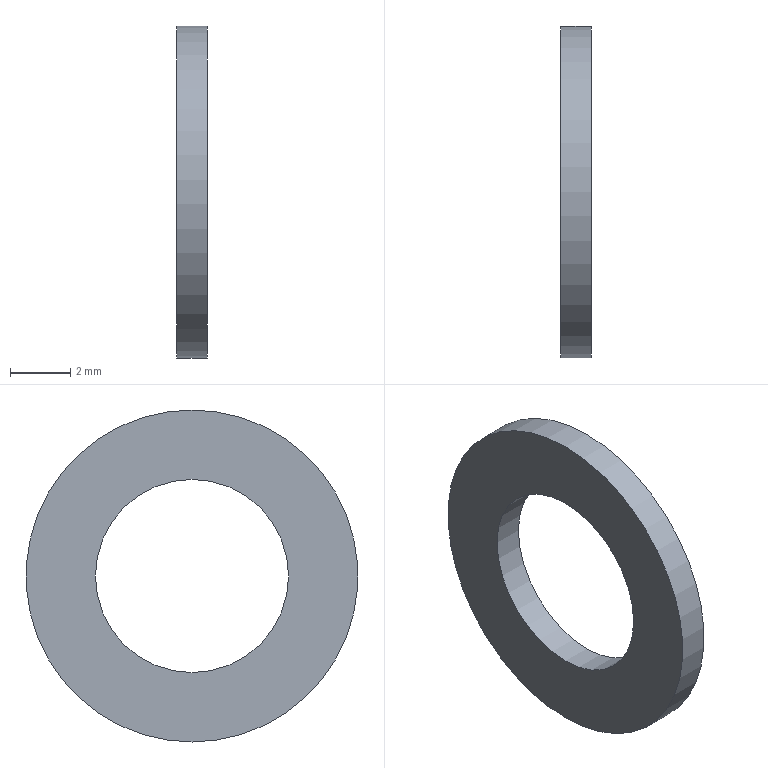Component | NX | ASSY_PRAC_PART_5 | 1 solid | 4 faces | box 1 x 11 x 11 mm | volume 63 mm3 | cylinder 2 | plane 2 | commonest cylinder face diameters 11 x1 6.4 x1
STEP:
#1=CARTESIAN_POINT('',(0.,0.,0.));
#2=DIRECTION('',(0.,0.,1.));
#3=DIRECTION('',(1.,0.,0.));
#4=AXIS2_PLACEMENT_3D('',#1,#2,#3);
#5=CARTESIAN_POINT('',(17.5,0.3851,26.061));
#6=VERTEX_POINT('',#5);
#7=CARTESIAN_POINT('',(17.5,0.3851,20.561));
#8=DIRECTION('',(-1.,0.,0.));
#9=DIRECTION('',(0.,0.,1.));
#10=AXIS2_PLACEMENT_3D('',#7,#8,#9);
#11=CIRCLE('',#10,5.5);
#12=CARTESIAN_POINT('',(17.5,0.3851,20.561));
#13=DIRECTION('',(1.,0.,0.));
#14=DIRECTION('',(0.,0.,-1.));
#15=AXIS2_PLACEMENT_3D('',#12,#13,#14);
#16=CYLINDRICAL_SURFACE('',#15,5.5);
#17=CARTESIAN_POINT('',(9.425,0.));
#18=DIRECTION('',(-1.,0.));
#19=VECTOR('',#18,1.);
#20=LINE('',#17,#19);
#21=(GEOMETRIC_REPRESENTATION_CONTEXT(2)PARAMETRIC_REPRESENTATION_CONTEXT()REPRESENTATION_CONTEXT('',''));
#22=DEFINITIONAL_REPRESENTATION('',(#20),#21);
#23=PCURVE('',#16,#22);
#24=CARTESIAN_POINT('',(17.5,0.3851,20.561));
#25=DIRECTION('',(-1.,0.,0.));
#26=DIRECTION('',(0.,0.,1.));
#27=AXIS2_PLACEMENT_3D('',#24,#25,#26);
#28=PLANE('',#27);
#29=CARTESIAN_POINT('',(0.,0.));
#30=DIRECTION('',(1.,0.));
#31=AXIS2_PLACEMENT_2D('',#29,#30);
#32=CIRCLE('',#31,5.5);
#33=(GEOMETRIC_REPRESENTATION_CONTEXT(2)PARAMETRIC_REPRESENTATION_CONTEXT()REPRESENTATION_CONTEXT('',''));
#34=DEFINITIONAL_REPRESENTATION('',(#32),#33);
#35=PCURVE('',#28,#34);
#36=SURFACE_CURVE('',#11,(#23,#35),.PCURVE_S1.);
#37=EDGE_CURVE('',#6,#6,#36,.T.);
#38=ORIENTED_EDGE('',*,*,#37,.F.);
#39=CARTESIAN_POINT('',(18.5,0.3851,26.061));
#40=VERTEX_POINT('',#39);
#41=CARTESIAN_POINT('',(17.5,0.3851,26.061));
#42=CARTESIAN_POINT('',(18.5,0.3851,26.061));
#43=B_SPLINE_CURVE_WITH_KNOTS('',1,(#41,#42),.UNSPECIFIED.,.F.,.F.,(2,2),(0.,1.),.PIECEWISE_BEZIER_KNOTS.);
#44=CARTESIAN_POINT('',(9.425,0.));
#45=DIRECTION('',(0.,1.));
#46=VECTOR('',#45,1.);
#47=LINE('',#44,#46);
#48=(GEOMETRIC_REPRESENTATION_CONTEXT(2)PARAMETRIC_REPRESENTATION_CONTEXT()REPRESENTATION_CONTEXT('',''));
#49=DEFINITIONAL_REPRESENTATION('',(#47),#48);
#50=PCURVE('',#16,#49);
#51=CARTESIAN_POINT('',(3.142,0.));
#52=DIRECTION('',(0.,1.));
#53=VECTOR('',#52,1.);
#54=LINE('',#51,#53);
#55=(GEOMETRIC_REPRESENTATION_CONTEXT(2)PARAMETRIC_REPRESENTATION_CONTEXT()REPRESENTATION_CONTEXT('',''));
#56=DEFINITIONAL_REPRESENTATION('',(#54),#55);
#57=PCURVE('',#16,#56);
#58=SEAM_CURVE('',#43,(#50,#57),.PCURVE_S1.);
#59=EDGE_CURVE('',#6,#40,#58,.T.);
#60=ORIENTED_EDGE('',*,*,#59,.T.);
#61=CARTESIAN_POINT('',(18.5,0.3851,20.561));
#62=DIRECTION('',(-1.,0.,0.));
#63=DIRECTION('',(0.,0.,1.));
#64=AXIS2_PLACEMENT_3D('',#61,#62,#63);
#65=CIRCLE('',#64,5.5);
#66=CARTESIAN_POINT('',(9.425,1.));
#67=DIRECTION('',(-1.,0.));
#68=VECTOR('',#67,1.);
#69=LINE('',#66,#68);
#70=(GEOMETRIC_REPRESENTATION_CONTEXT(2)PARAMETRIC_REPRESENTATION_CONTEXT()REPRESENTATION_CONTEXT('',''));
#71=DEFINITIONAL_REPRESENTATION('',(#69),#70);
#72=PCURVE('',#16,#71);
#73=CARTESIAN_POINT('',(18.5,0.3851,20.561));
#74=DIRECTION('',(-1.,0.,0.));
#75=DIRECTION('',(0.,0.,1.));
#76=AXIS2_PLACEMENT_3D('',#73,#74,#75);
#77=PLANE('',#76);
#78=CARTESIAN_POINT('',(0.,0.));
#79=DIRECTION('',(1.,0.));
#80=AXIS2_PLACEMENT_2D('',#78,#79);
#81=CIRCLE('',#80,5.5);
#82=(GEOMETRIC_REPRESENTATION_CONTEXT(2)PARAMETRIC_REPRESENTATION_CONTEXT()REPRESENTATION_CONTEXT('',''));
#83=DEFINITIONAL_REPRESENTATION('',(#81),#82);
#84=PCURVE('',#77,#83);
#85=SURFACE_CURVE('',#65,(#72,#84),.PCURVE_S1.);
#86=EDGE_CURVE('',#40,#40,#85,.T.);
#87=ORIENTED_EDGE('',*,*,#86,.T.);
#88=ORIENTED_EDGE('',*,*,#59,.F.);
#89=EDGE_LOOP('',(#38,#60,#87,#88));
#90=FACE_BOUND('',#89,.T.);
#91=ADVANCED_FACE('',(#90),#16,.T.);
#92=CARTESIAN_POINT('',(17.5,0.3851,23.761));
#93=VERTEX_POINT('',#92);
#94=CARTESIAN_POINT('',(17.5,0.3851,20.561));
#95=DIRECTION('',(-1.,0.,0.));
#96=DIRECTION('',(0.,0.,1.));
#97=AXIS2_PLACEMENT_3D('',#94,#95,#96);
#98=CIRCLE('',#97,3.2);
#99=CARTESIAN_POINT('',(17.5,0.3851,20.561));
#100=DIRECTION('',(1.,0.,0.));
#101=DIRECTION('',(0.,0.,-1.));
#102=AXIS2_PLACEMENT_3D('',#99,#100,#101);
#103=CYLINDRICAL_SURFACE('',#102,3.2);
#104=CARTESIAN_POINT('',(9.425,0.));
#105=DIRECTION('',(-1.,0.));
#106=VECTOR('',#105,1.);
#107=LINE('',#104,#106);
#108=(GEOMETRIC_REPRESENTATION_CONTEXT(2)PARAMETRIC_REPRESENTATION_CONTEXT()REPRESENTATION_CONTEXT('',''));
#109=DEFINITIONAL_REPRESENTATION('',(#107),#108);
#110=PCURVE('',#103,#109);
#111=CARTESIAN_POINT('',(0.,0.));
#112=DIRECTION('',(1.,0.));
#113=AXIS2_PLACEMENT_2D('',#111,#112);
#114=CIRCLE('',#113,3.2);
#115=(GEOMETRIC_REPRESENTATION_CONTEXT(2)PARAMETRIC_REPRESENTATION_CONTEXT()REPRESENTATION_CONTEXT('',''));
#116=DEFINITIONAL_REPRESENTATION('',(#114),#115);
#117=PCURVE('',#28,#116);
#118=SURFACE_CURVE('',#98,(#110,#117),.PCURVE_S1.);
#119=EDGE_CURVE('',#93,#93,#118,.T.);
#120=ORIENTED_EDGE('',*,*,#119,.F.);
#121=CARTESIAN_POINT('',(18.5,0.3851,23.761));
#122=VERTEX_POINT('',#121);
#123=CARTESIAN_POINT('',(17.5,0.3851,23.761));
#124=CARTESIAN_POINT('',(18.5,0.3851,23.761));
#125=B_SPLINE_CURVE_WITH_KNOTS('',1,(#123,#124),.UNSPECIFIED.,.F.,.F.,(2,2),(0.,1.),.PIECEWISE_BEZIER_KNOTS.);
#126=CARTESIAN_POINT('',(9.425,0.));
#127=DIRECTION('',(0.,1.));
#128=VECTOR('',#127,1.);
#129=LINE('',#126,#128);
#130=(GEOMETRIC_REPRESENTATION_CONTEXT(2)PARAMETRIC_REPRESENTATION_CONTEXT()REPRESENTATION_CONTEXT('',''));
#131=DEFINITIONAL_REPRESENTATION('',(#129),#130);
#132=PCURVE('',#103,#131);
#133=CARTESIAN_POINT('',(3.142,0.));
#134=DIRECTION('',(0.,1.));
#135=VECTOR('',#134,1.);
#136=LINE('',#133,#135);
#137=(GEOMETRIC_REPRESENTATION_CONTEXT(2)PARAMETRIC_REPRESENTATION_CONTEXT()REPRESENTATION_CONTEXT('',''));
#138=DEFINITIONAL_REPRESENTATION('',(#136),#137);
#139=PCURVE('',#103,#138);
#140=SEAM_CURVE('',#125,(#132,#139),.PCURVE_S1.);
#141=EDGE_CURVE('',#93,#122,#140,.T.);
#142=ORIENTED_EDGE('',*,*,#141,.T.);
#143=CARTESIAN_POINT('',(18.5,0.3851,20.561));
#144=DIRECTION('',(-1.,0.,0.));
#145=DIRECTION('',(0.,0.,1.));
#146=AXIS2_PLACEMENT_3D('',#143,#144,#145);
#147=CIRCLE('',#146,3.2);
#148=CARTESIAN_POINT('',(9.425,1.));
#149=DIRECTION('',(-1.,0.));
#150=VECTOR('',#149,1.);
#151=LINE('',#148,#150);
#152=(GEOMETRIC_REPRESENTATION_CONTEXT(2)PARAMETRIC_REPRESENTATION_CONTEXT()REPRESENTATION_CONTEXT('',''));
#153=DEFINITIONAL_REPRESENTATION('',(#151),#152);
#154=PCURVE('',#103,#153);
#155=CARTESIAN_POINT('',(0.,0.));
#156=DIRECTION('',(1.,0.));
#157=AXIS2_PLACEMENT_2D('',#155,#156);
#158=CIRCLE('',#157,3.2);
#159=(GEOMETRIC_REPRESENTATION_CONTEXT(2)PARAMETRIC_REPRESENTATION_CONTEXT()REPRESENTATION_CONTEXT('',''));
#160=DEFINITIONAL_REPRESENTATION('',(#158),#159);
#161=PCURVE('',#77,#160);
#162=SURFACE_CURVE('',#147,(#154,#161),.PCURVE_S1.);
#163=EDGE_CURVE('',#122,#122,#162,.T.);
#164=ORIENTED_EDGE('',*,*,#163,.T.);
#165=ORIENTED_EDGE('',*,*,#141,.F.);
#166=EDGE_LOOP('',(#120,#142,#164,#165));
#167=FACE_BOUND('',#166,.F.);
#168=ADVANCED_FACE('',(#167),#103,.F.);
#169=ORIENTED_EDGE('',*,*,#37,.T.);
#170=EDGE_LOOP('',(#169));
#171=FACE_BOUND('',#170,.T.);
#172=ORIENTED_EDGE('',*,*,#119,.F.);
#173=EDGE_LOOP('',(#172));
#174=FACE_BOUND('',#173,.T.);
#175=ADVANCED_FACE('',(#171,#174),#28,.T.);
#176=ORIENTED_EDGE('',*,*,#86,.F.);
#177=EDGE_LOOP('',(#176));
#178=FACE_BOUND('',#177,.T.);
#179=ORIENTED_EDGE('',*,*,#163,.T.);
#180=EDGE_LOOP('',(#179));
#181=FACE_BOUND('',#180,.T.);
#182=ADVANCED_FACE('',(#178,#181),#77,.F.);
#183=CLOSED_SHELL('',(#91,#168,#175,#182));
#184=MANIFOLD_SOLID_BREP('',#183);
#185=(LENGTH_UNIT()NAMED_UNIT(*)SI_UNIT(.MILLI.,.METRE.));
#186=UNCERTAINTY_MEASURE_WITH_UNIT(LENGTH_MEASURE(0.00001),#185,'','');
#187=(NAMED_UNIT(*)PLANE_ANGLE_UNIT()SI_UNIT($,.RADIAN.));
#188=(NAMED_UNIT(*)SI_UNIT($,.STERADIAN.)SOLID_ANGLE_UNIT());
#189=(GEOMETRIC_REPRESENTATION_CONTEXT(3)GLOBAL_UNCERTAINTY_ASSIGNED_CONTEXT((#186))GLOBAL_UNIT_ASSIGNED_CONTEXT((#185,#187,#188))REPRESENTATION_CONTEXT('',''));
#190=ADVANCED_BREP_SHAPE_REPRESENTATION('',(#4,#184),#189);